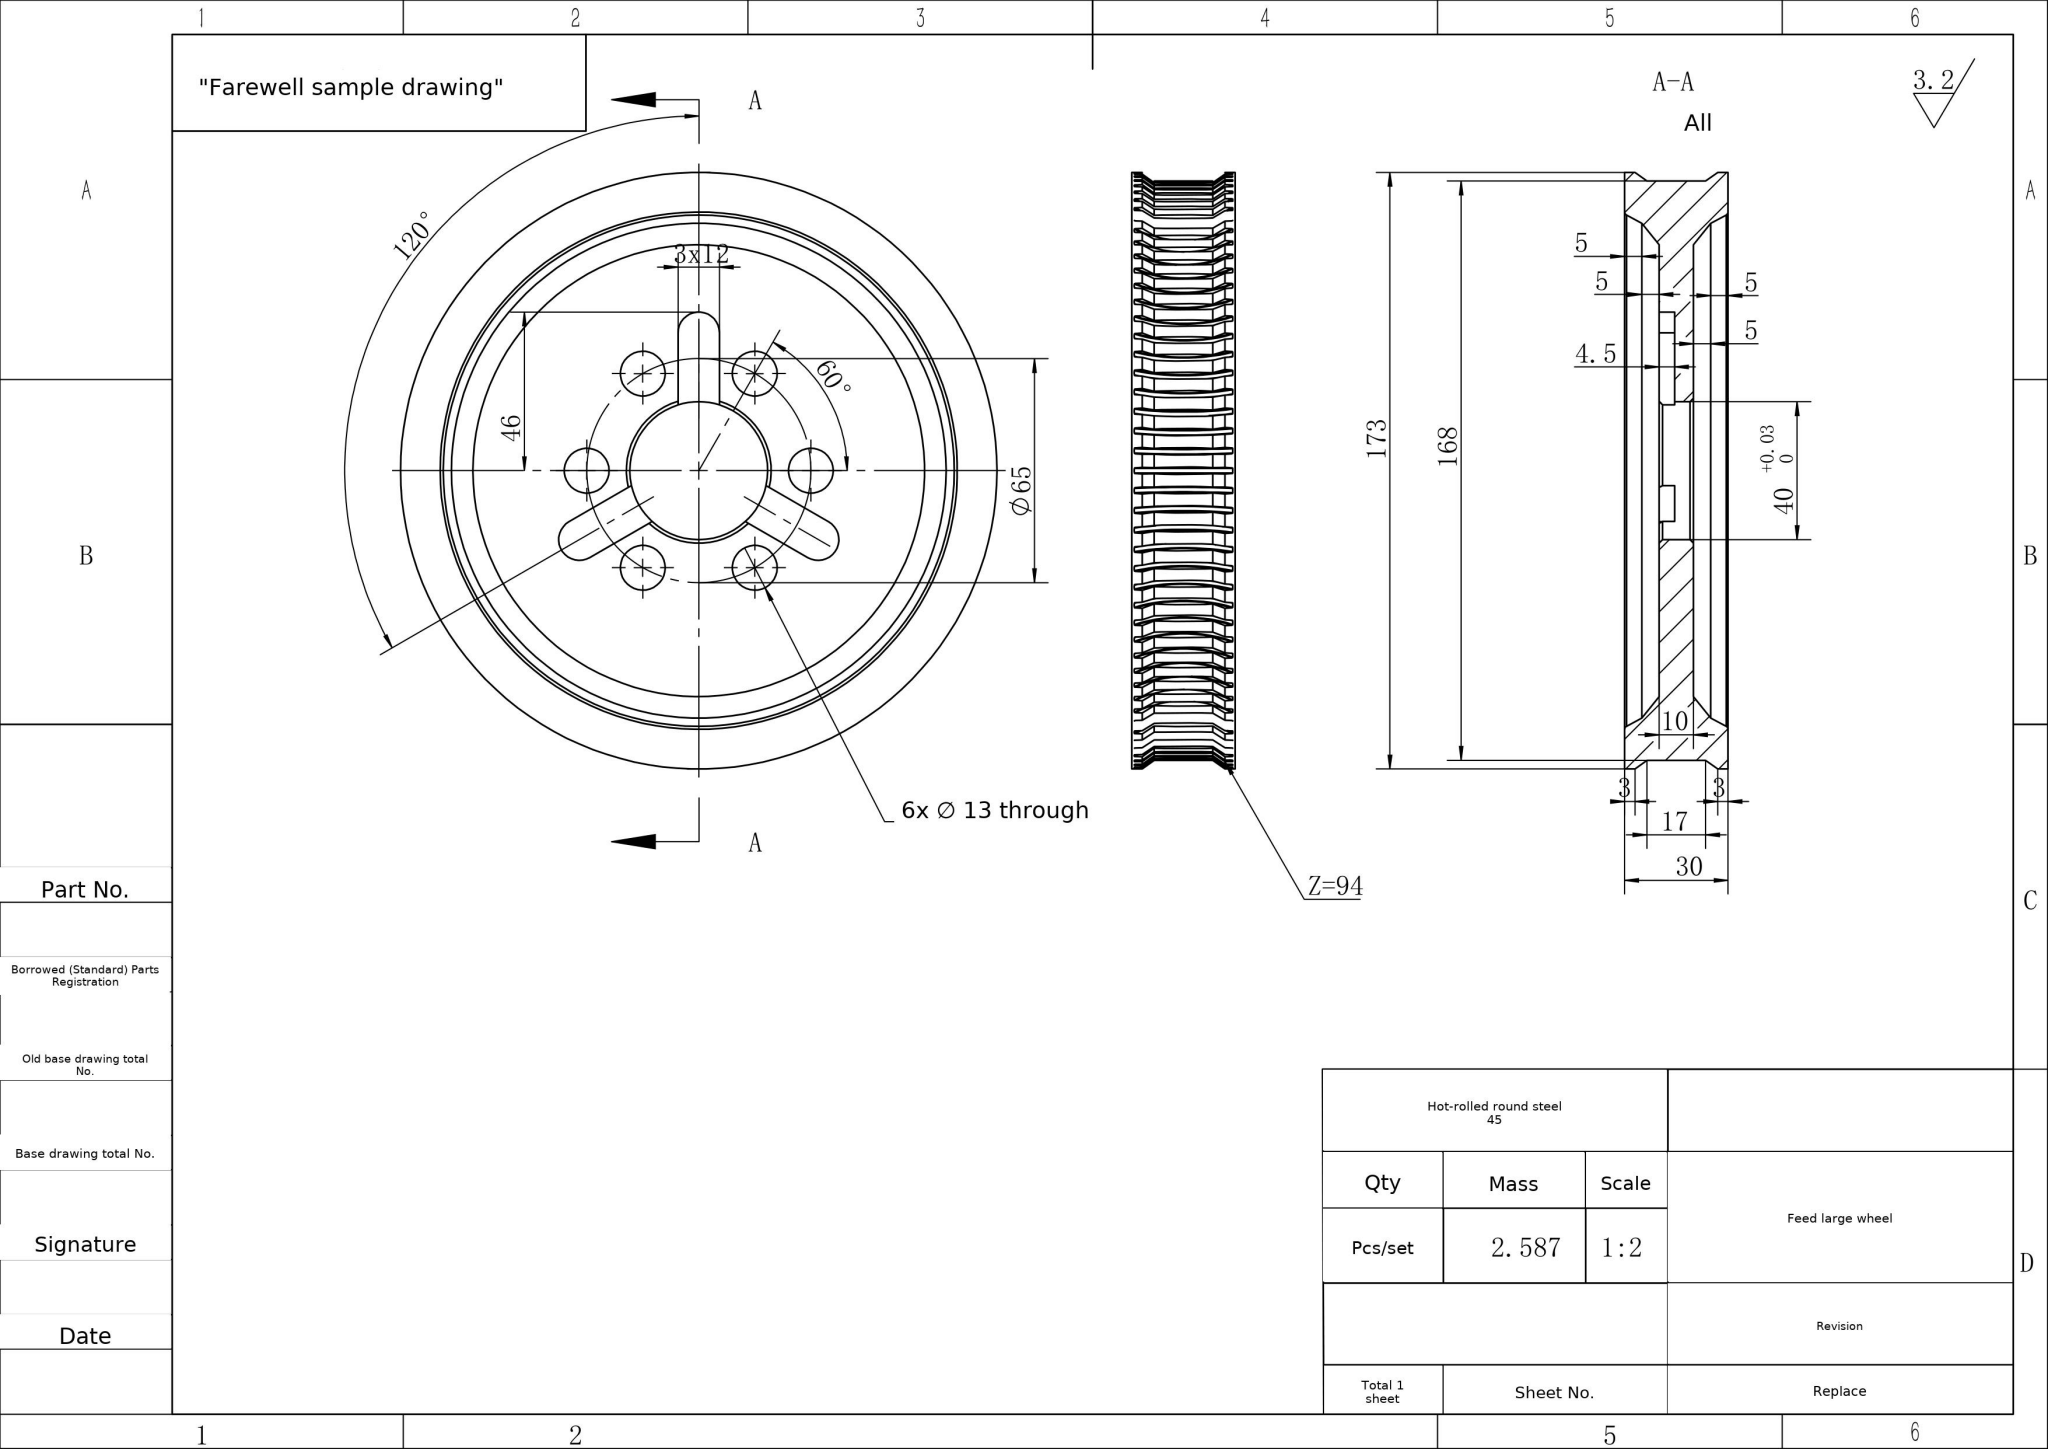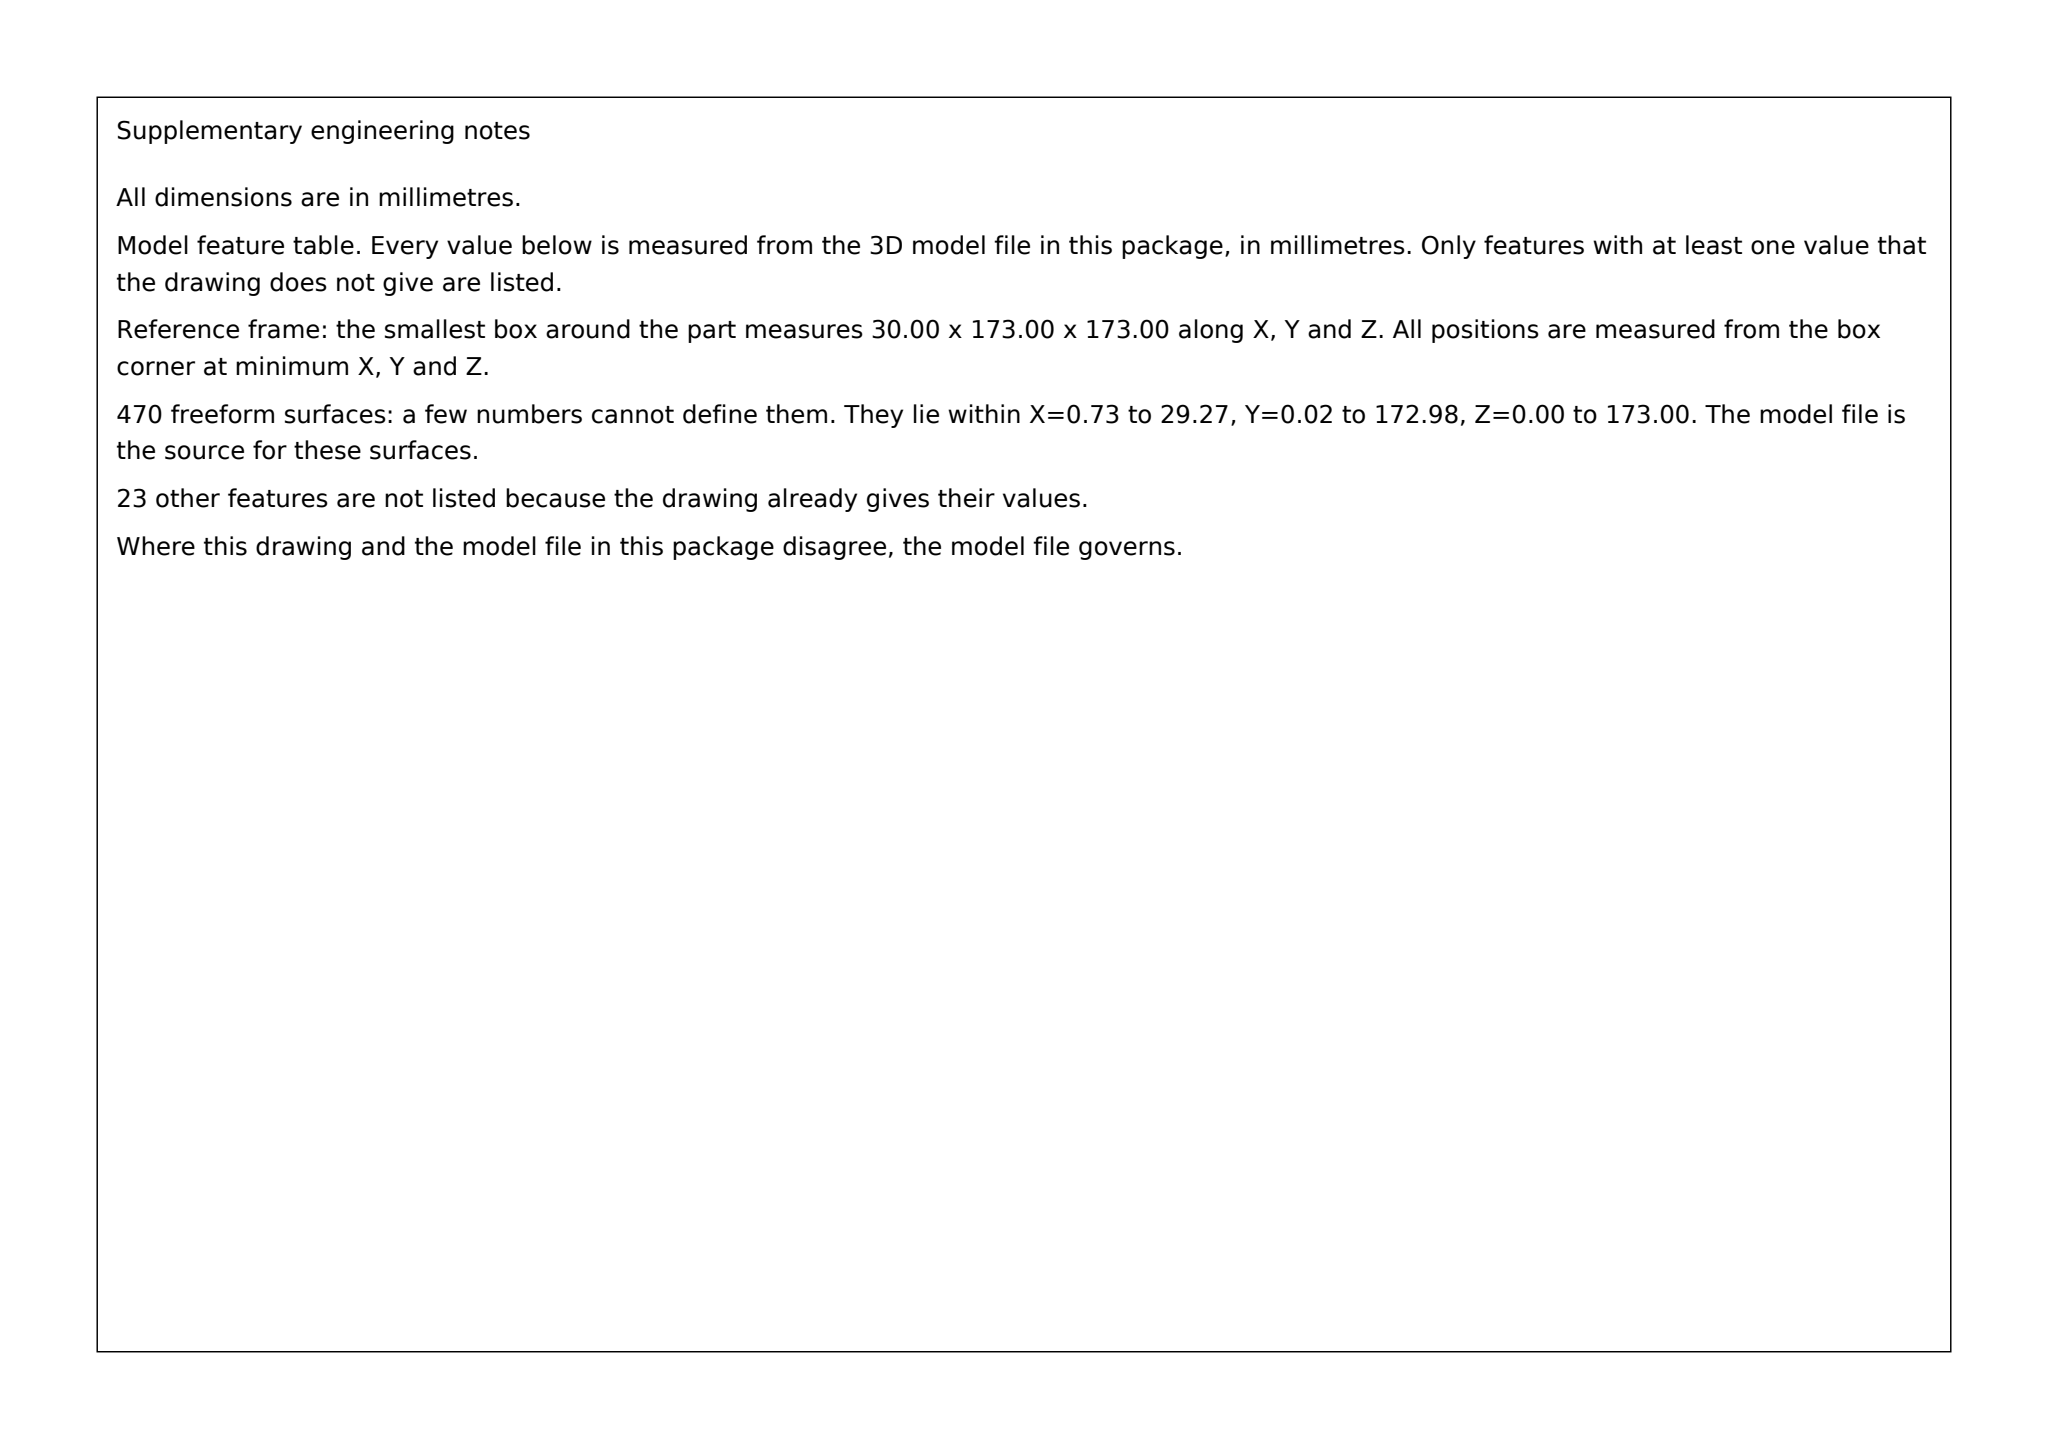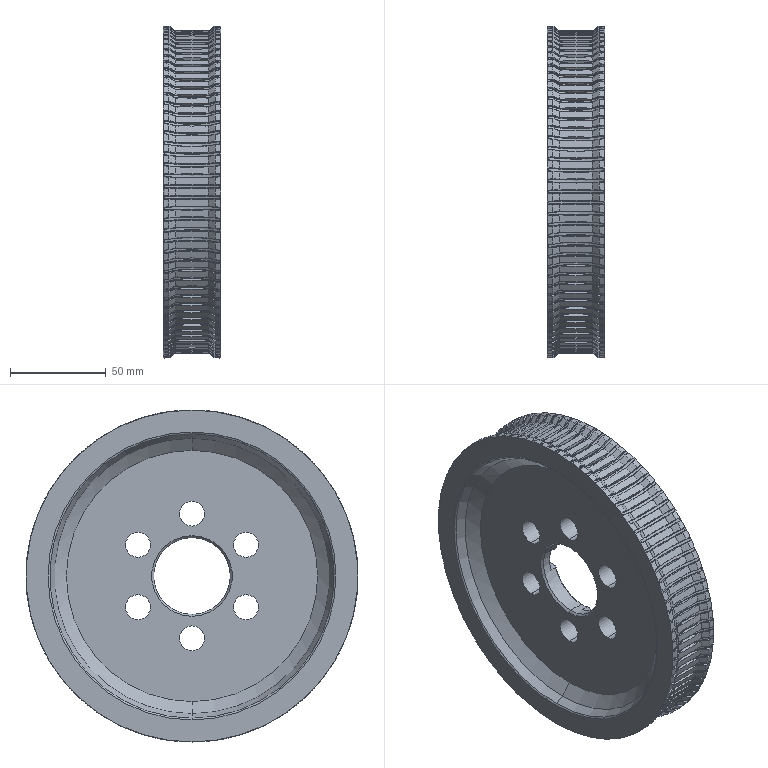Part | SolidWorks | mm | material Hot-rolled round steel 45 | 1 solid | 805 faces | box 30 x 173 x 173 mm | volume 331694 mm3 | spline 470 | cone 202 | cylinder 116 | plane 13 | torus 4 | commonest cylinder face diameters 168 x94 13 x12 12 x4 173 x4 40 x2